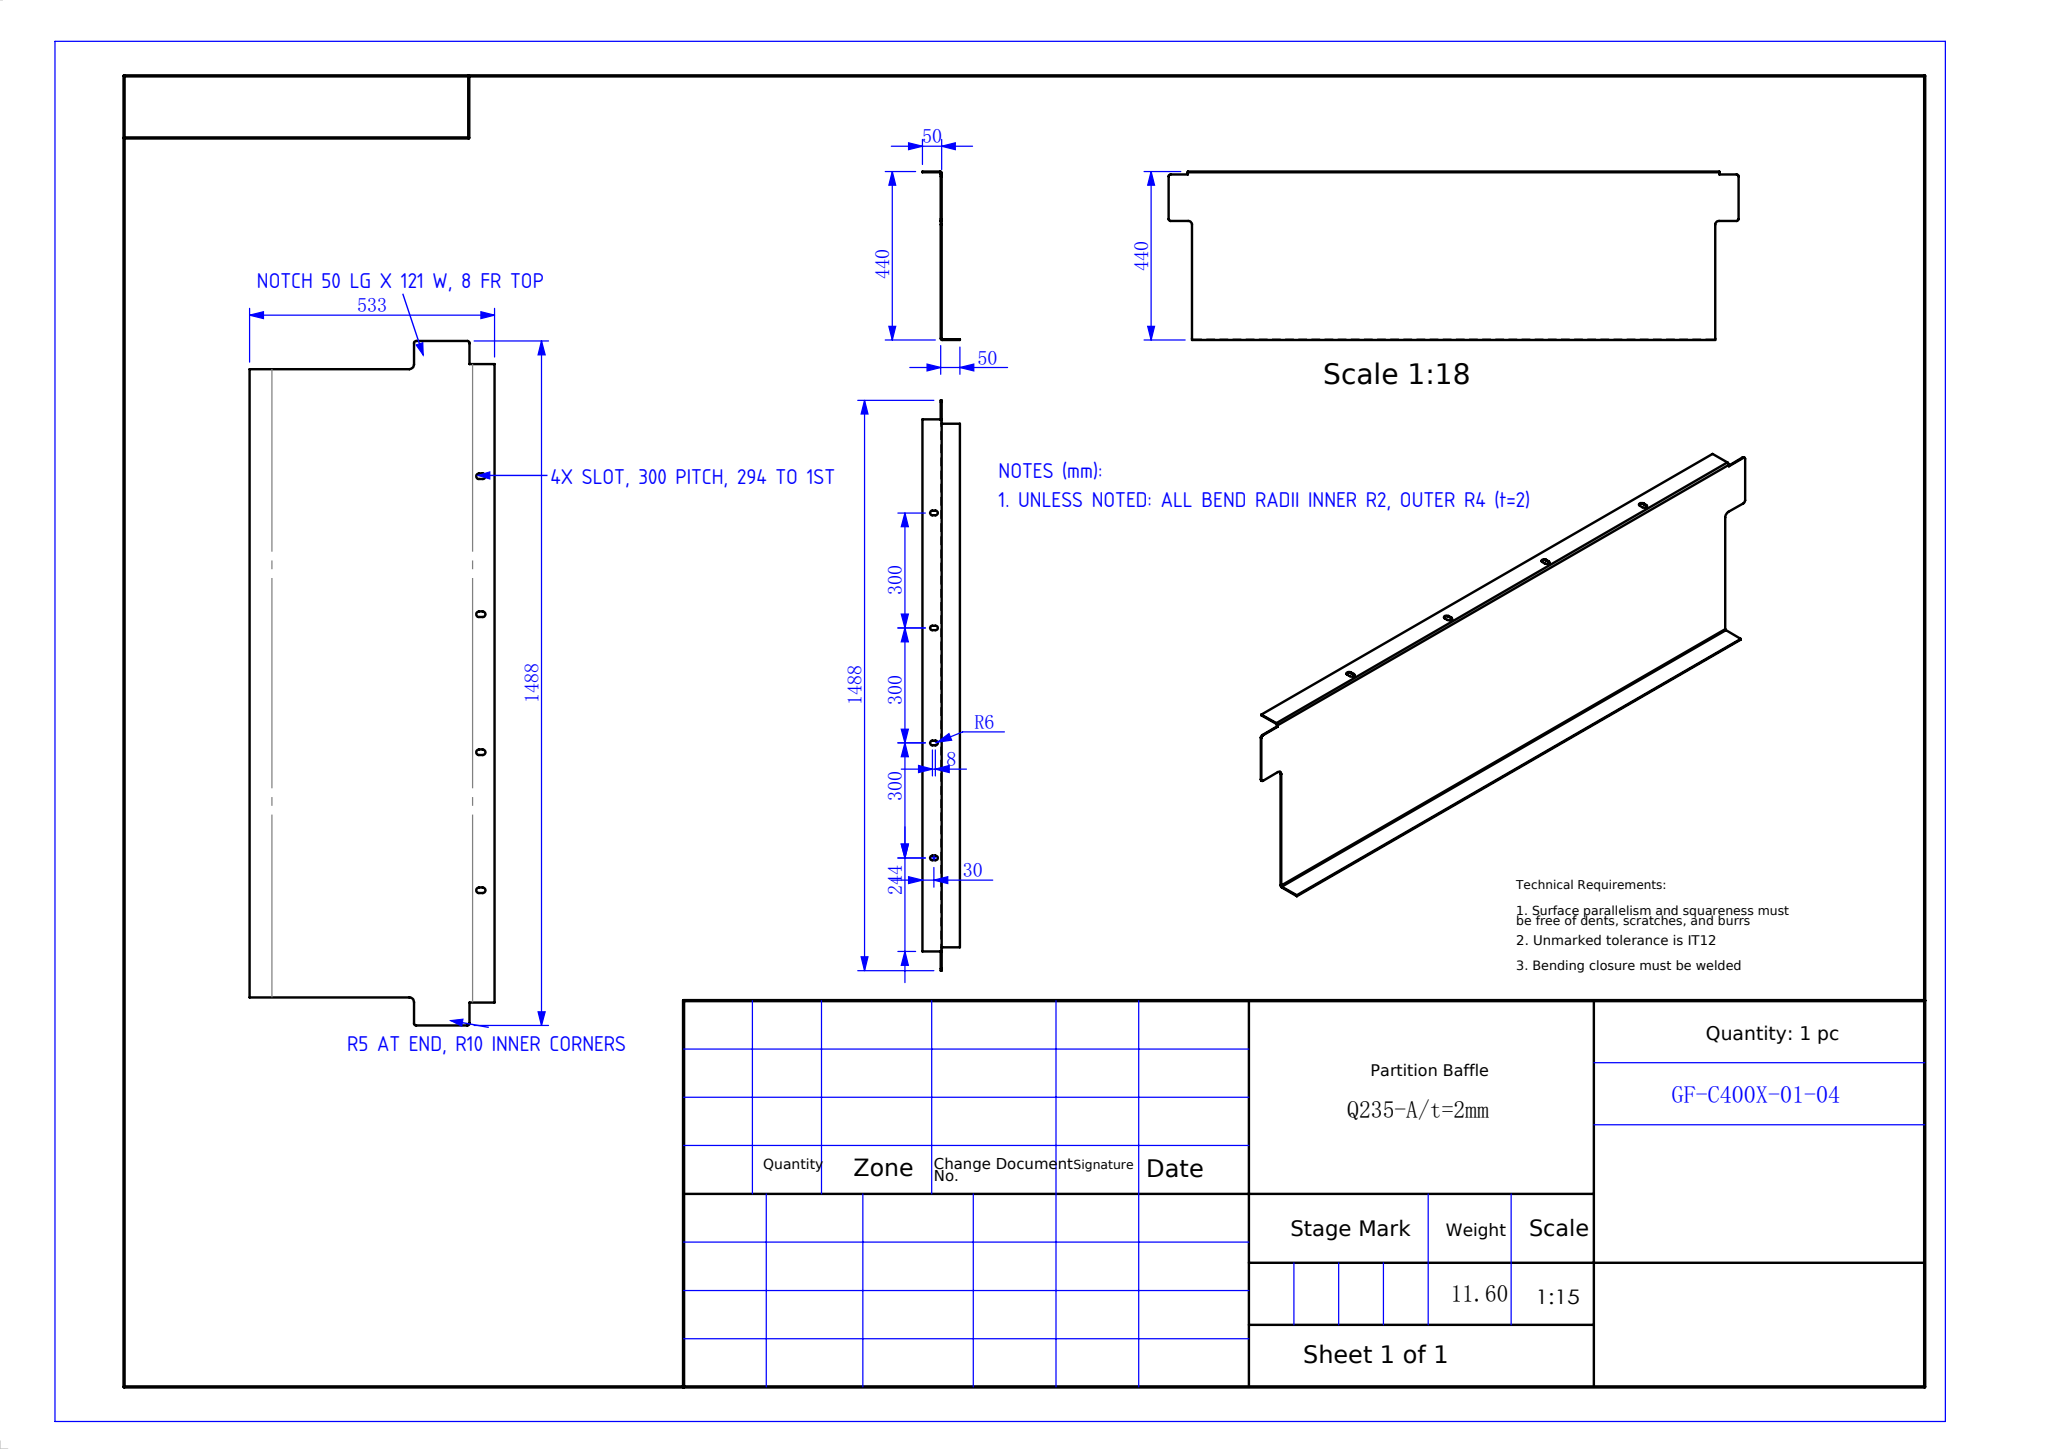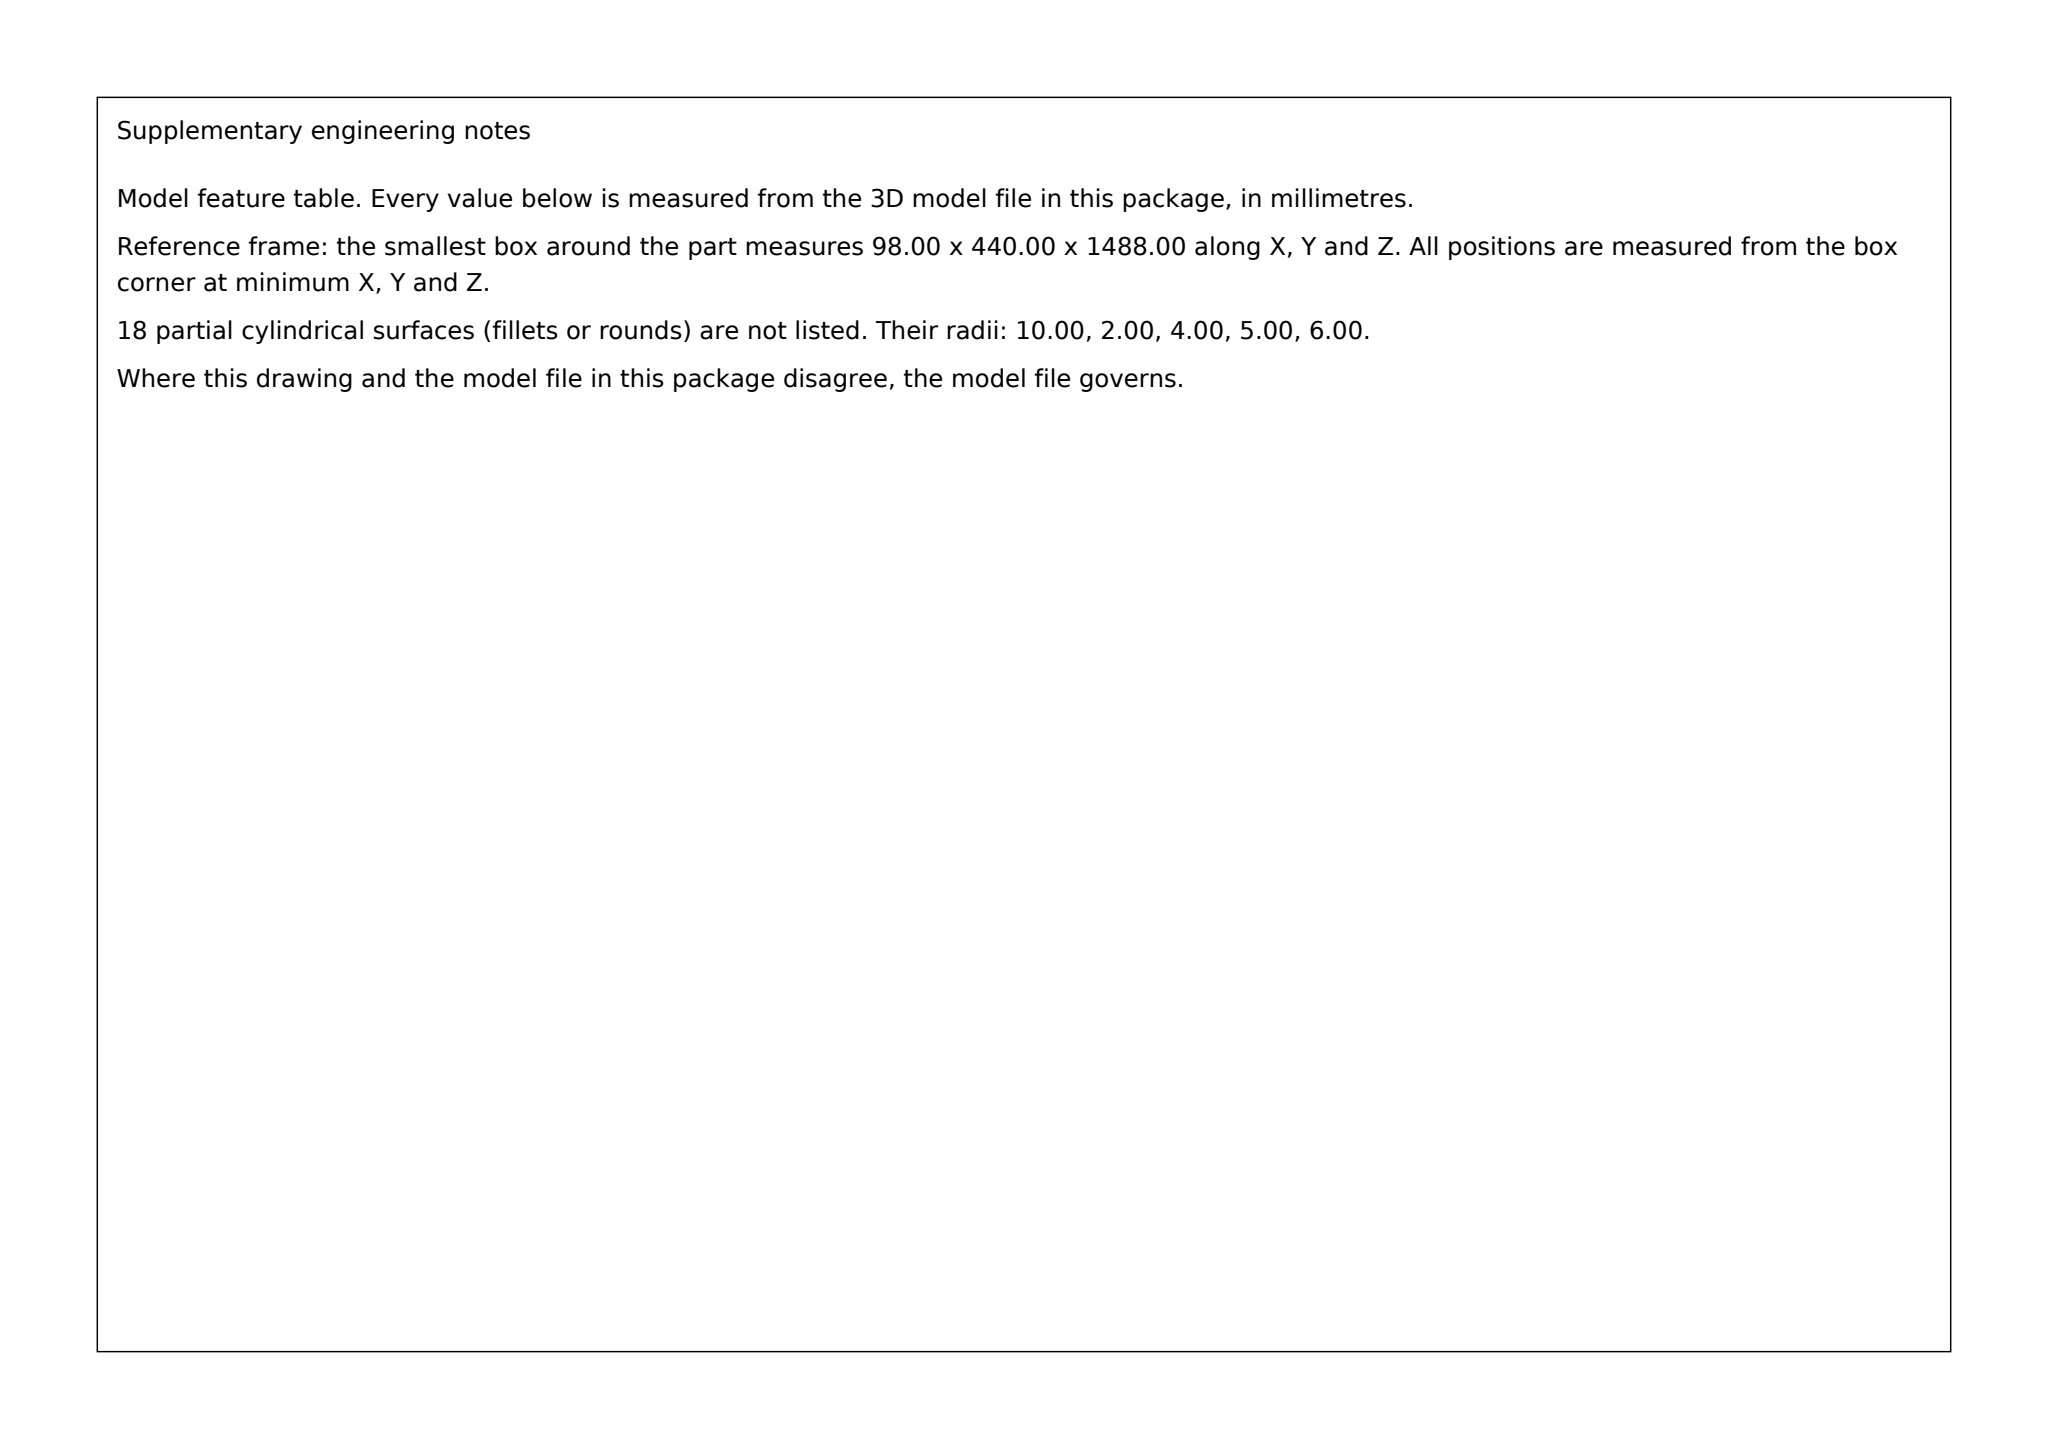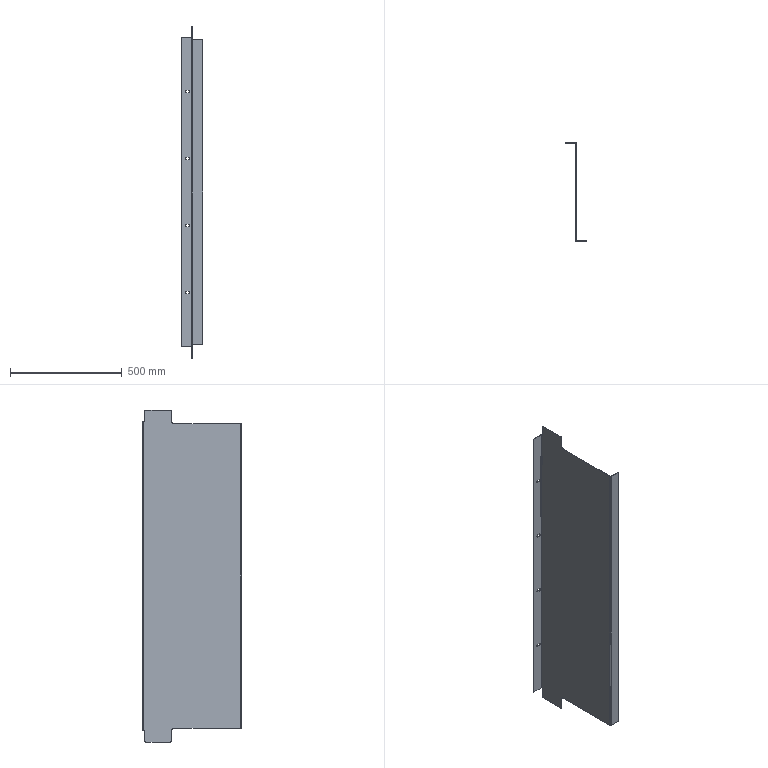Part | SolidWorks | mm | material Q235-A | 1 solid | 48 faces | box 98 x 440 x 1488 mm | volume 1487618 mm3 | plane 26 | cylinder 22 | commonest cylinder face diameters 12 x12 10 x4 4 x2 8 x2 20 x2
Drawing notes:
END NOTCH BOTH ENDS: 50 LG x 121 WIDE, 8 FROM TOP EDGE | from the solid: z planes 0/50 & 1438/1488; y planes 311 & 432 (x2); bbox y=440 (440-432=8, 432-311=121)
END NOTCH CORNERS: R5 AT PART END, R10 AT INNER CORNERS | from the solid: x-axis cyl D10 at (y316,z5),(y427,z5),(y316,z1483),(y427,z1483) = R5; x-axis cyl D20 at (y301,z51),(y301,z1437) = R10
4 SLOTS @ 300 PITCH, FIRST CL 294 FROM END OF PART | from the solid: y-axis D12 slot cyls at z=294,594,894,1194; bbox z=1488 gives 294 at each end
UNLESS NOTED: ALL BEND RADII INNER R2, OUTER R4 (t=2) | from the solid: Web/flange faces at x=0,2 and x=48,50,98 with t=2 sheet; web-to-flange bends give inner R2 / outer R4 per STEP